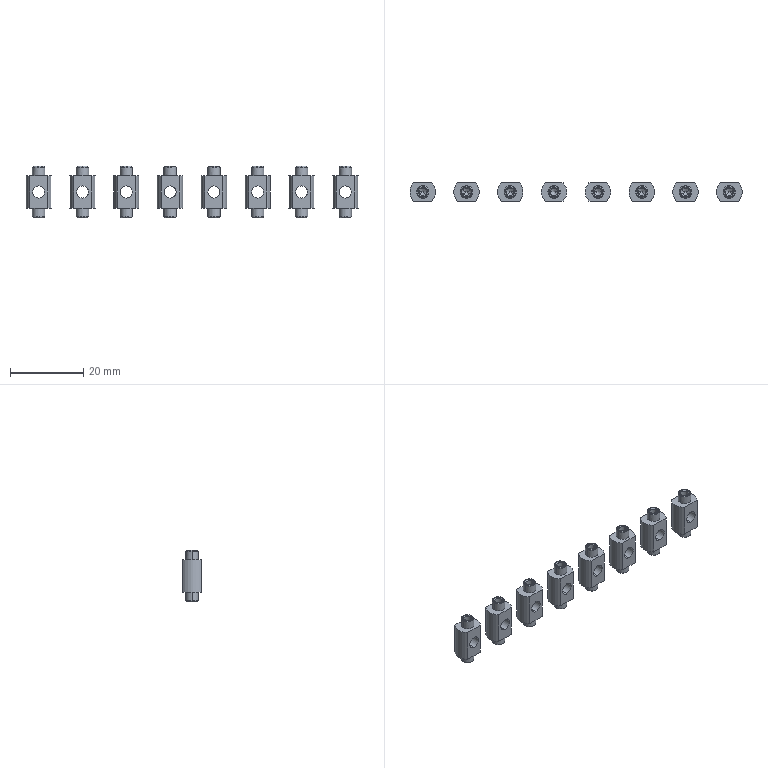CAM job | Mastercam | mm | 22 operations | part box 91 x 5 x 14
1. 3D High Speed (Dynamic OptiRough) | 2 - 10C
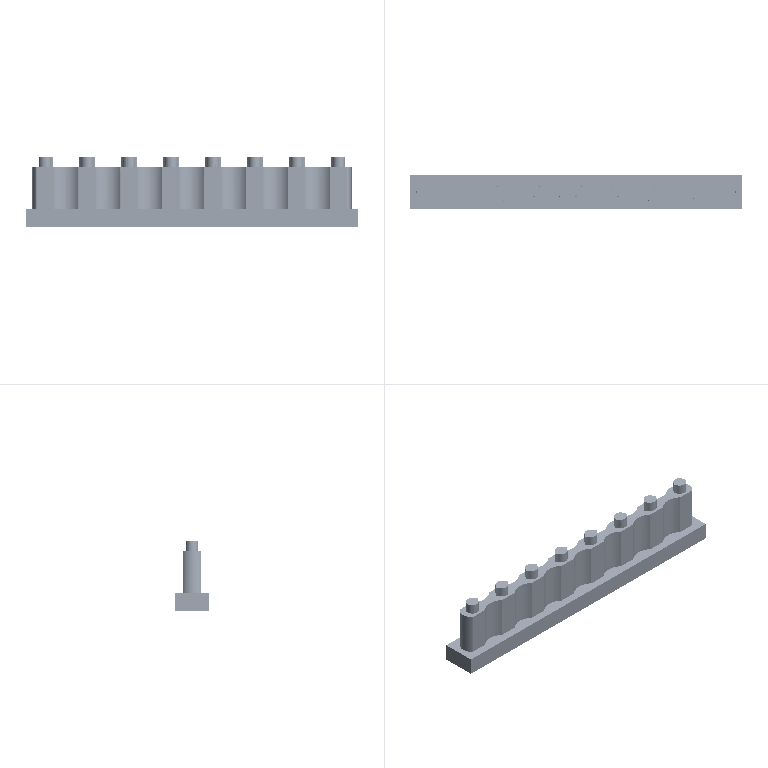2. 3D High Speed (Waterline rest passes) | 4 - 4C
3. Drill/Counterbore | 6 - 6 倒角刀
4. Peck Drill | 29 - 2.1 钻头
5. Facing | 3 - 10J
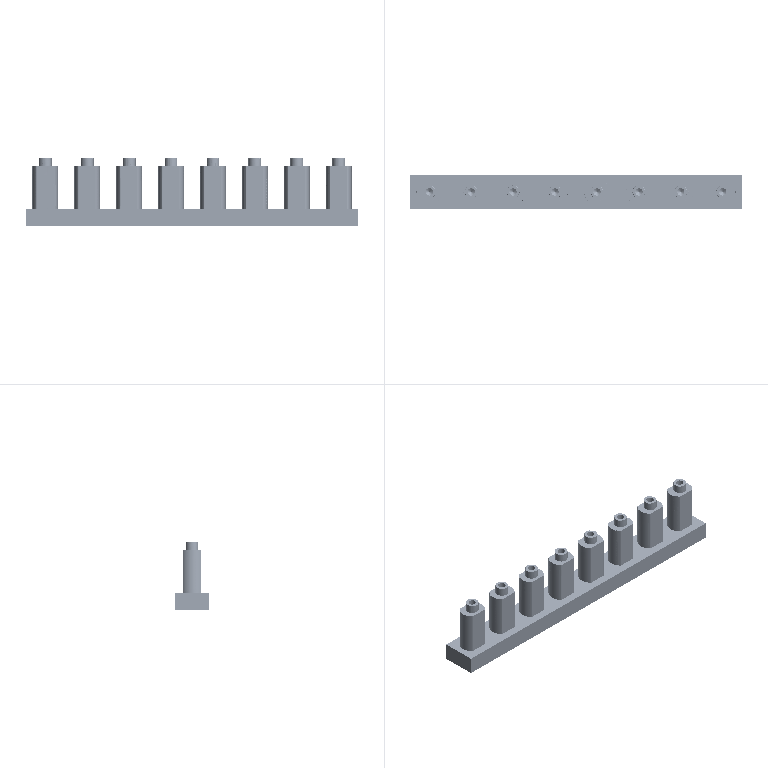6. Contour (2D) | 5 - 4J
7. Contour (2D) | 5 - 4J
8. Chamfer Drill | 6 - 6 倒角刀
9. Contour (2D chamfer) | 6 - 6 倒角刀
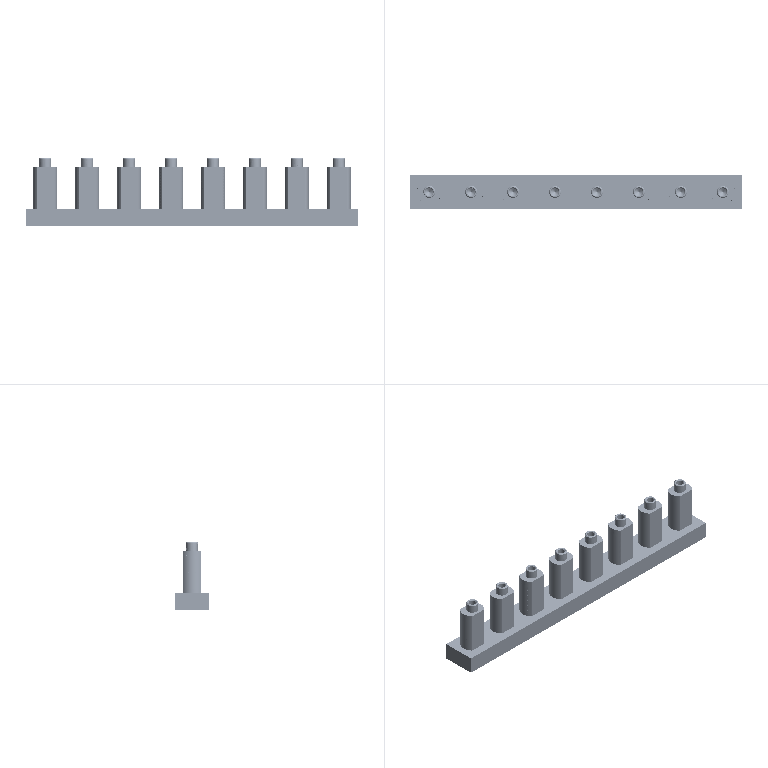10. Contour (2D chamfer) | 11 - 4 倒角刀
11. Drill/Counterbore | 6 - 6 倒角刀
12. Peck Drill | 17 - 3.3 钻头
13. Chamfer Drill | 6 - 6 倒角刀
14. Facing | 2 - 10C
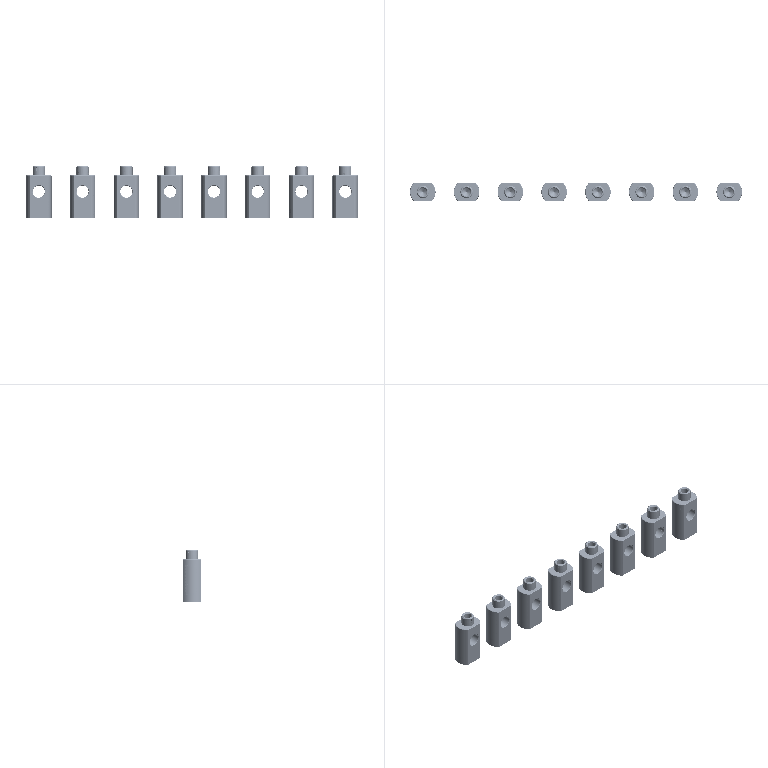15. Facing | 3 - 10J
16. Contour (Ramp) | 4 - 4C
17. Contour (2D) | 5 - 4J
18. Drill/Counterbore | 11 - 4 倒角刀
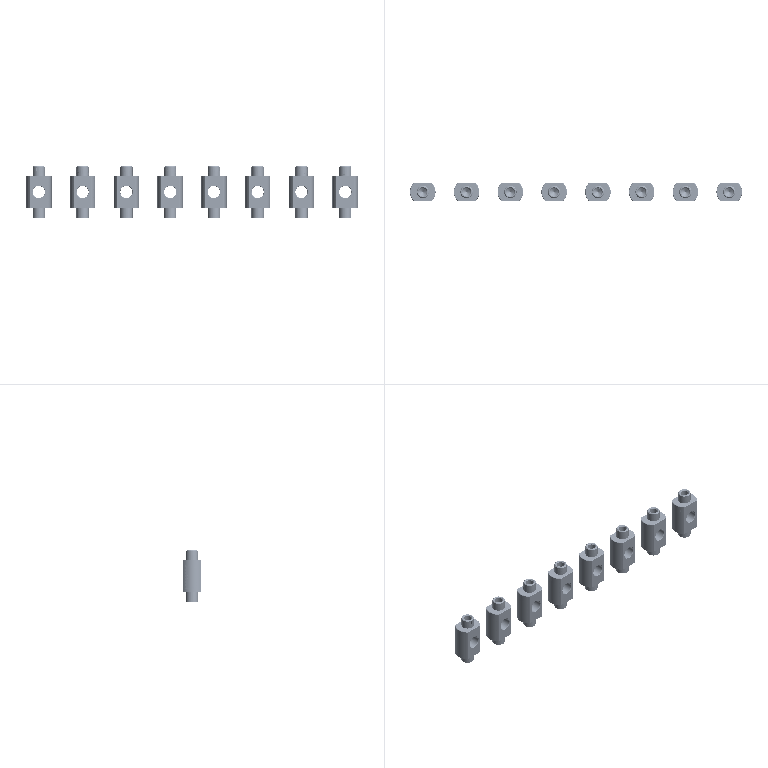19. Peck Drill | 29 - 2.1 钻头
20. Chamfer Drill | 11 - 4 倒角刀
21. Contour (2D chamfer) | 11 - 4 倒角刀
22. Contour (2D chamfer) | 11 - 4 倒角刀